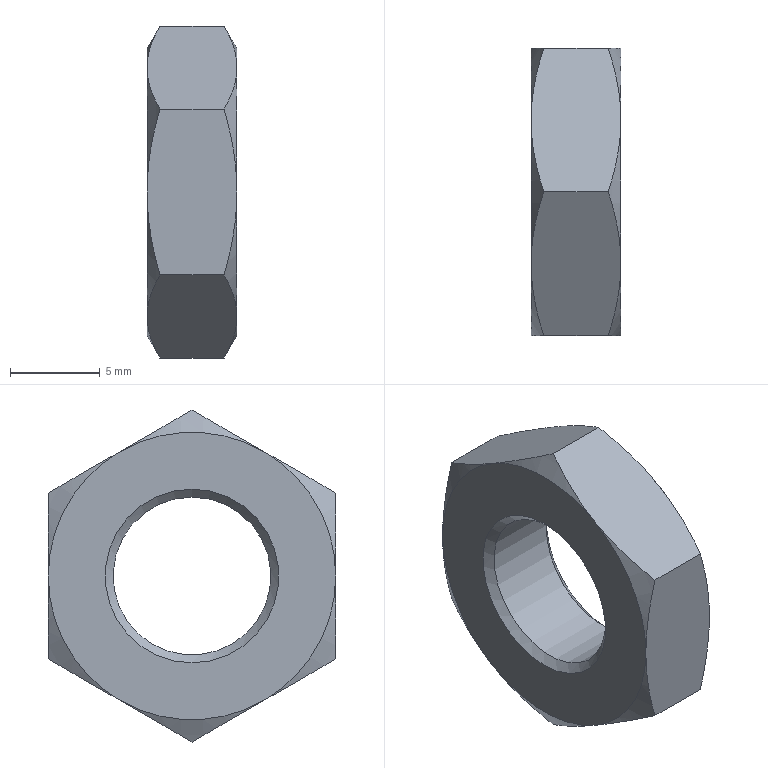Component | NX | GB-T6172_1-2000_M10X1_5_2 | 1 solid | 23 faces | volume 791 mm3 | cone 14 | plane 8 | cylinder 1 | commonest cylinder face diameters 8.782 x1